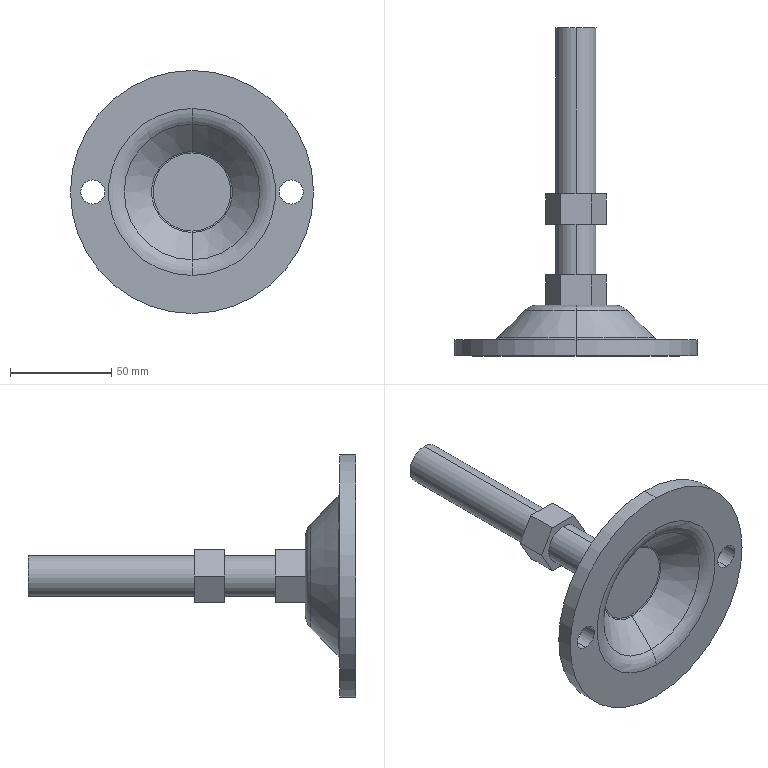Component | SolidWorks | BF-20AdjustableCupFoot-1 | 3 solids | 45 faces | box 120 x 162 x 120 mm | volume 149607 mm3 | plane 21 | cylinder 12 | torus 8 | cone 4 | commonest cylinder face diameters 20 x6 12 x4 120 x2 | material Q235A
build123d program:
from build123d import *

# Parameters (mm, degrees)
SKETCH1_W           = 10
SKETCH1_H           = 137
SKETCH3_R           = 10
BOSS_EXTRUDE2_DEPTH = 15
LPATTERN1_COUNT     = 2
LPATTERN1_PITCH     = 40
SKETCH4_R           = 6
CUT_EXTRUDE1_DEPTH  = 176.829


with BuildPart() as part:
    # Sketch1 → Revolve1 (revolve)
    with BuildSketch(Plane.XY, mode=Mode.PRIVATE) as revolve1_sk:
        with BuildLine():
            Line((19.979, 16.707), (33.464, 3.222))
            ThreePointArc((33.464, 3.222), (37.033, 0.8373), (41.243, 0))
            Line((41.243, 0), (60, 0))
            Line((60, 0), (60, 8))
            Line((60, 8), (41.243, 8))
            ThreePointArc((41.243, 8), (40.095, 8.228), (39.121, 8.879))
            Line((39.121, 8.879), (25.636, 22.364))
            ThreePointArc((25.636, 22.364), (22.716, 24.315), (19.272, 25))
            Line((19.272, 25), (0, 25))
            Line((0, 25), (0, 17))
            Line((0, 17), (19.272, 17))
            ThreePointArc((19.272, 17), (19.655, 16.924), (19.979, 16.707))
        make_face()
        with Locations((5, 93.5)):
            Rectangle(SKETCH1_W, SKETCH1_H)
    revolve(revolve1_sk.sketch.rotate(Axis((0, 25, 0), (0, 1, 0)), 90), axis=Axis((0, 25, 0), (0, 1, 0)))

    # Sketch4 → Cut-Extrude1 (cut, through all)
    with BuildSketch(Plane(origin=(0, 8, 0), x_dir=(1, 0, 0), z_dir=(0, 1, 0))):
        with Locations(Location((-49, 0, 0), (0, 0, 270))):
            Circle(SKETCH4_R)
        with Locations(Location((49, 0, 0), (0, 0, 270))):
            Circle(SKETCH4_R)
    extrude(amount=-CUT_EXTRUDE1_DEPTH, mode=Mode.SUBTRACT)


with BuildPart() as body_2:
    # Sketch3 → Boss-Extrude2 (new body)
    with BuildSketch(Plane(origin=(0, 25, 0), x_dir=(1, 0, 0), z_dir=(0, 1, 0))):
        Polygon((7.506, 13), (-7.506, 13), (-15.011, 0), (-7.506, -13), (7.506, -13), (15.011, 0), align=None)
        with Locations(Location((0, 0, 0), (0, 0, 270))):
            Circle(SKETCH3_R, mode=Mode.SUBTRACT)
    extrude(amount=BOSS_EXTRUDE2_DEPTH)


with BuildPart() as lpattern1_1:
    # LPattern1: pattern copy
    add(body_2.part.moved(Location(Vector(0, 1, 0) * (1 * LPATTERN1_PITCH))))


solid = Compound([part.part, body_2.part, lpattern1_1.part])

# Placed as in the assembly
solid = solid.moved(Location((-144.116, -435.633, 342.9), (0, 0, 0)))